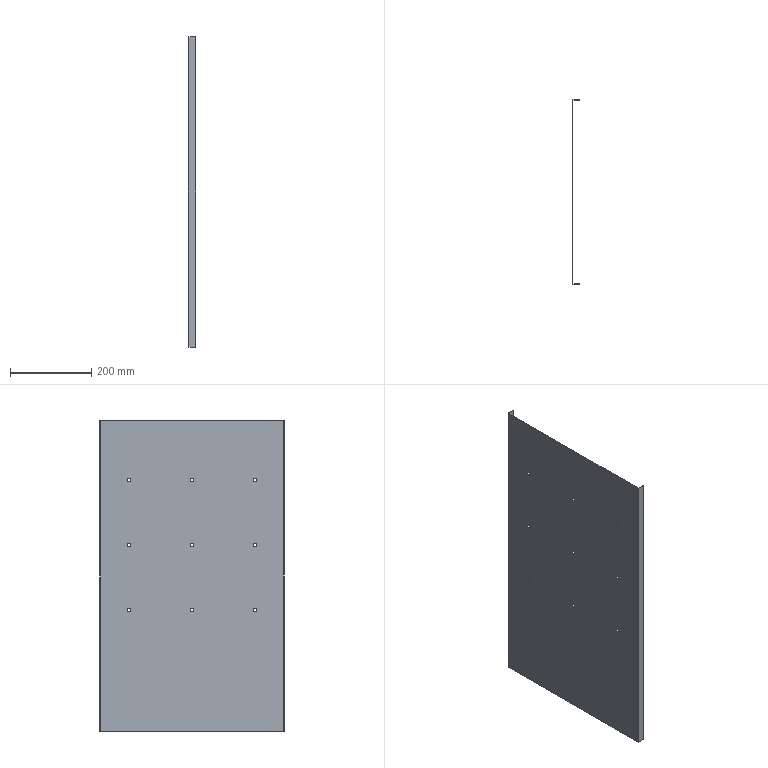Component | SolidWorks | UpperLeftSidePlate-1_UpperLeftOuterSidePanelInnerPanel-2_UpperLeftOuterSidePanelInnerPanel-1 | 1 solid | 40 faces | volume 300792 mm3 | cylinder 22 | plane 18 | commonest cylinder face diameters 8 x18 3.6 x2 2 x2 | material 304